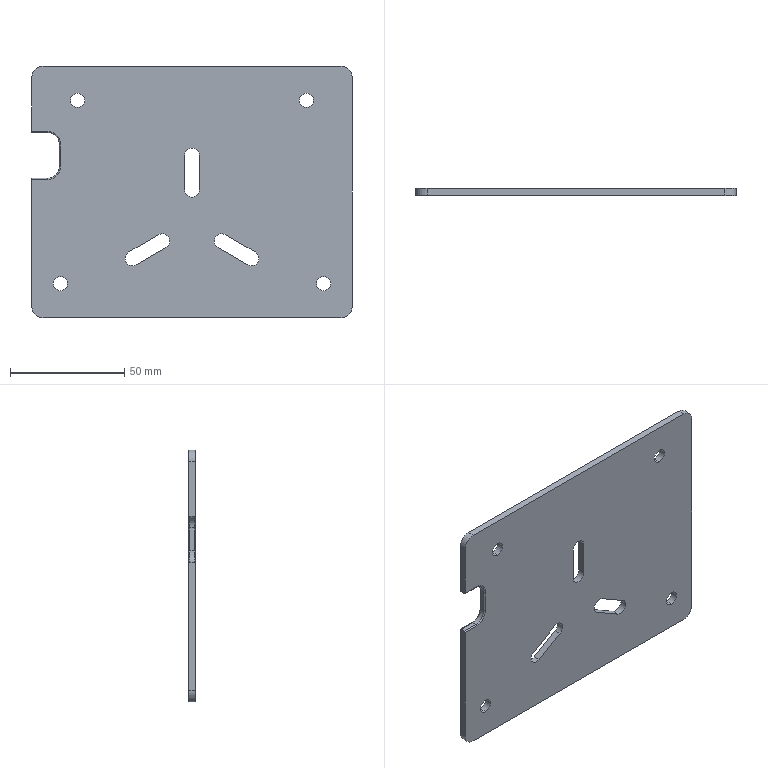CAM job | Mastercam | mm | 4 operations | part box 140 x 3 x 110
1. Contour (Ramp) | 4 - 4 平铣刀
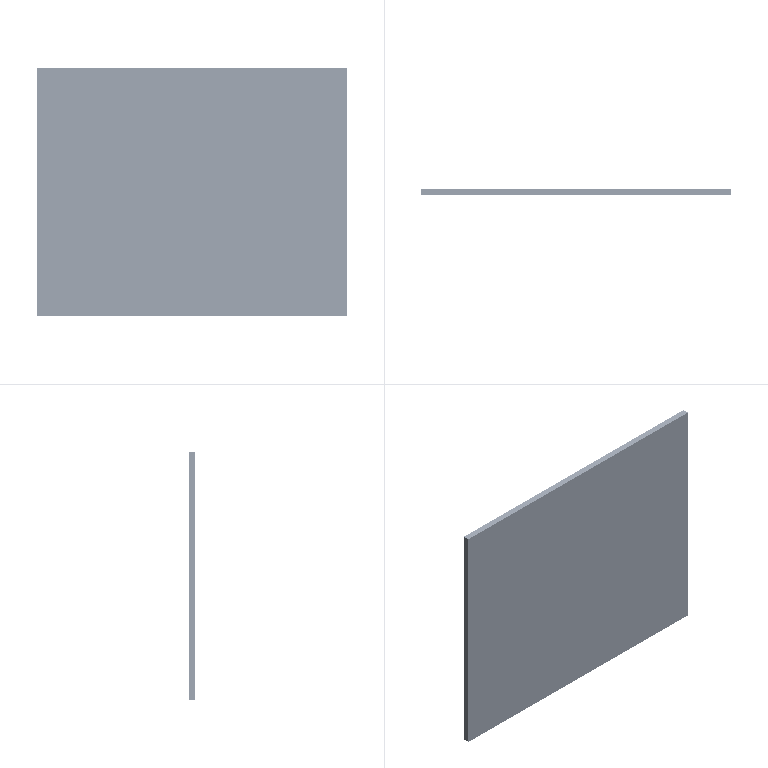2. Drill/Counterbore | 7 - 4 倒角刀
3. Contour (2D) | 2 - 2 平铣刀
4. Contour (2D chamfer) | 7 - 4 倒角刀